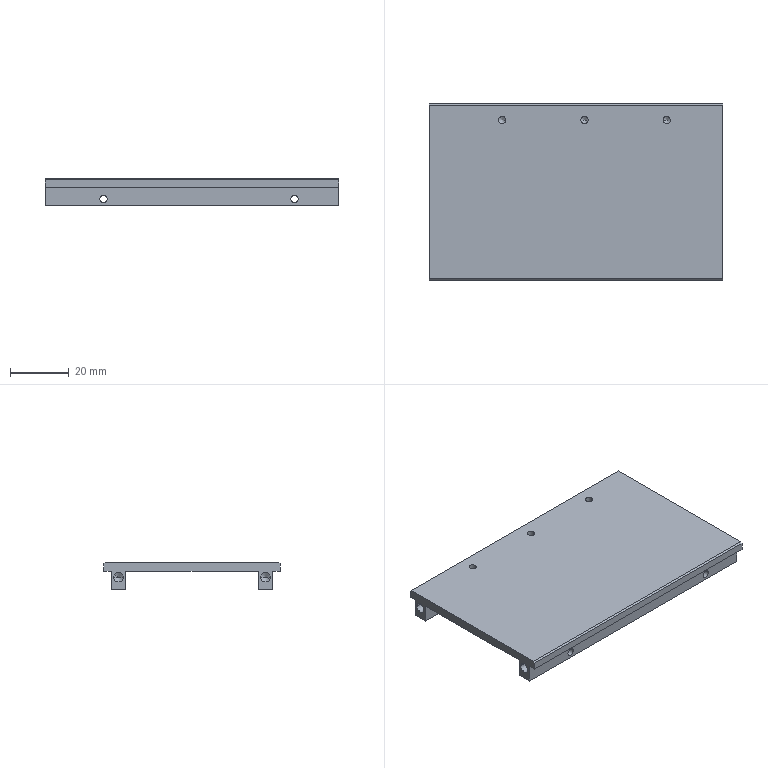CAM job | Mastercam | mm | 12 operations | part box 99.75 x 60 x 11.59
1. Drill/Counterbore | 1 - 6 倒角刀
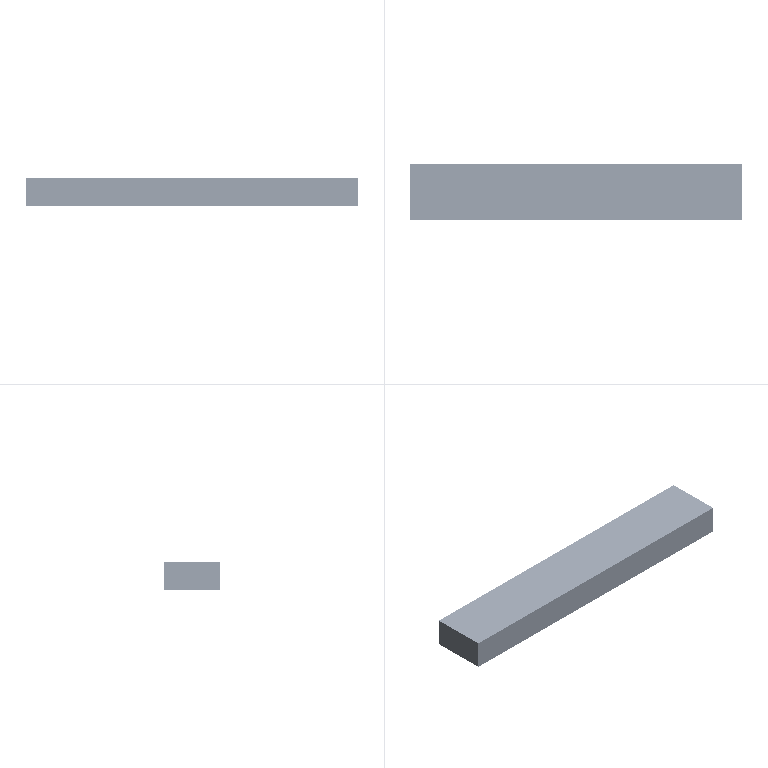2. Peck Drill | 11 - 3.3 钻头
3. Chamfer Drill | 1 - 6 倒角刀
4. Drill/Counterbore | 1 - 6 倒角刀
5. Peck Drill | 7 - 2.5 钻头
6. Chamfer Drill | 1 - 6 倒角刀
7. Drill/Counterbore | 1 - 6 倒角刀
8. Peck Drill | 7 - 2.5 钻头
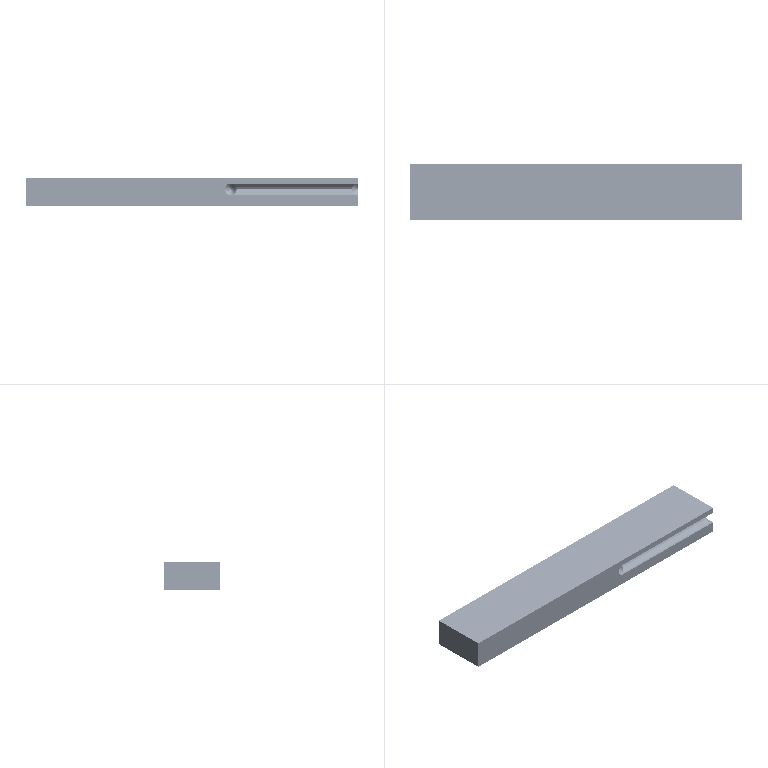9. Chamfer Drill | 1 - 6 倒角刀
10. Drill/Counterbore | 1 - 6 倒角刀
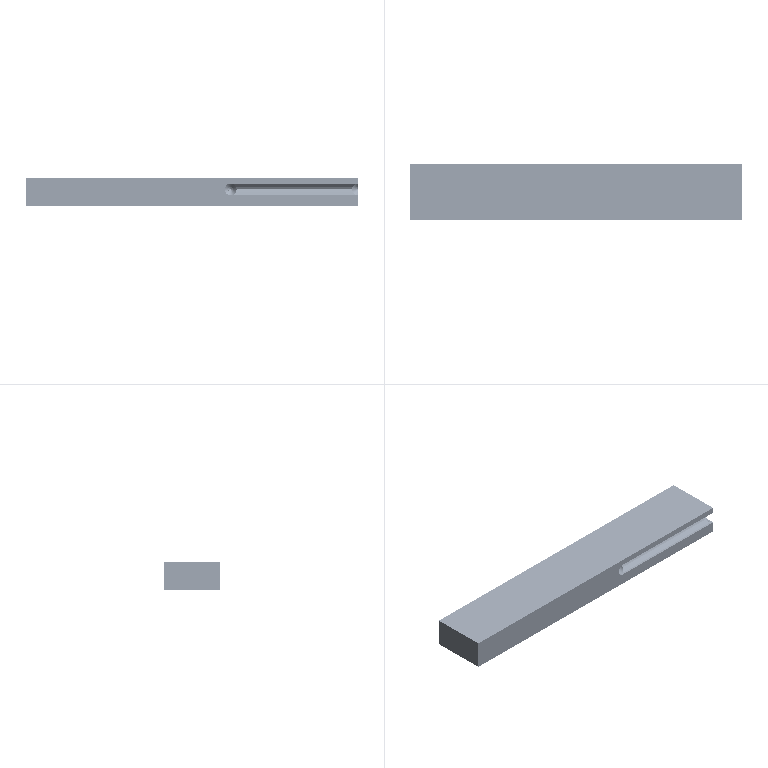11. Peck Drill | 7 - 2.5 钻头
12. Chamfer Drill | 1 - 6 倒角刀